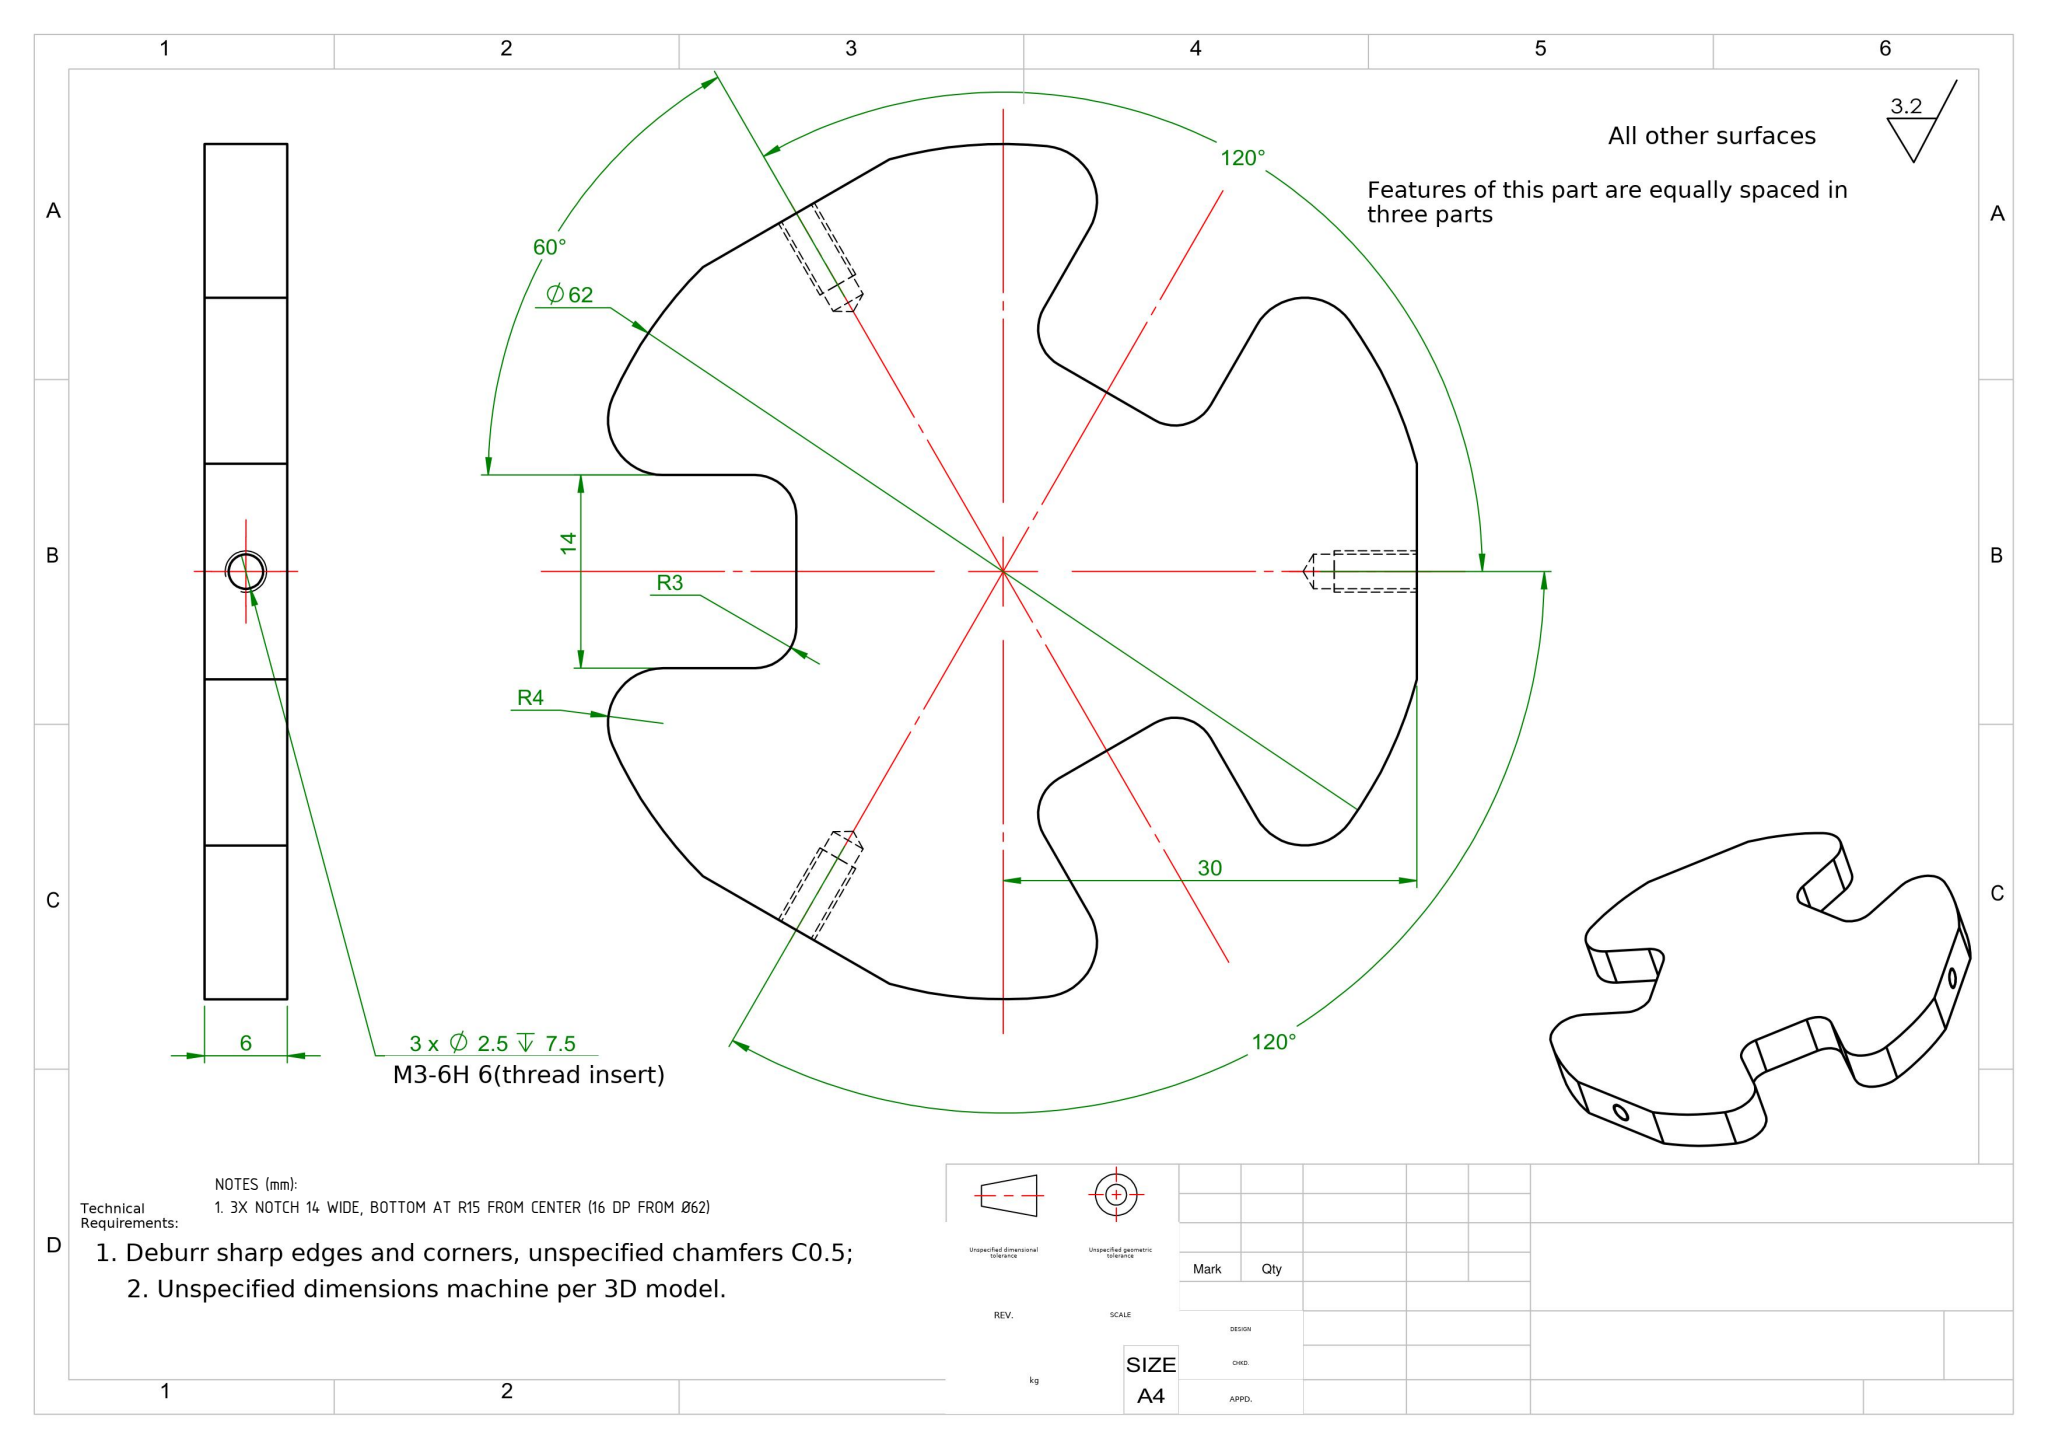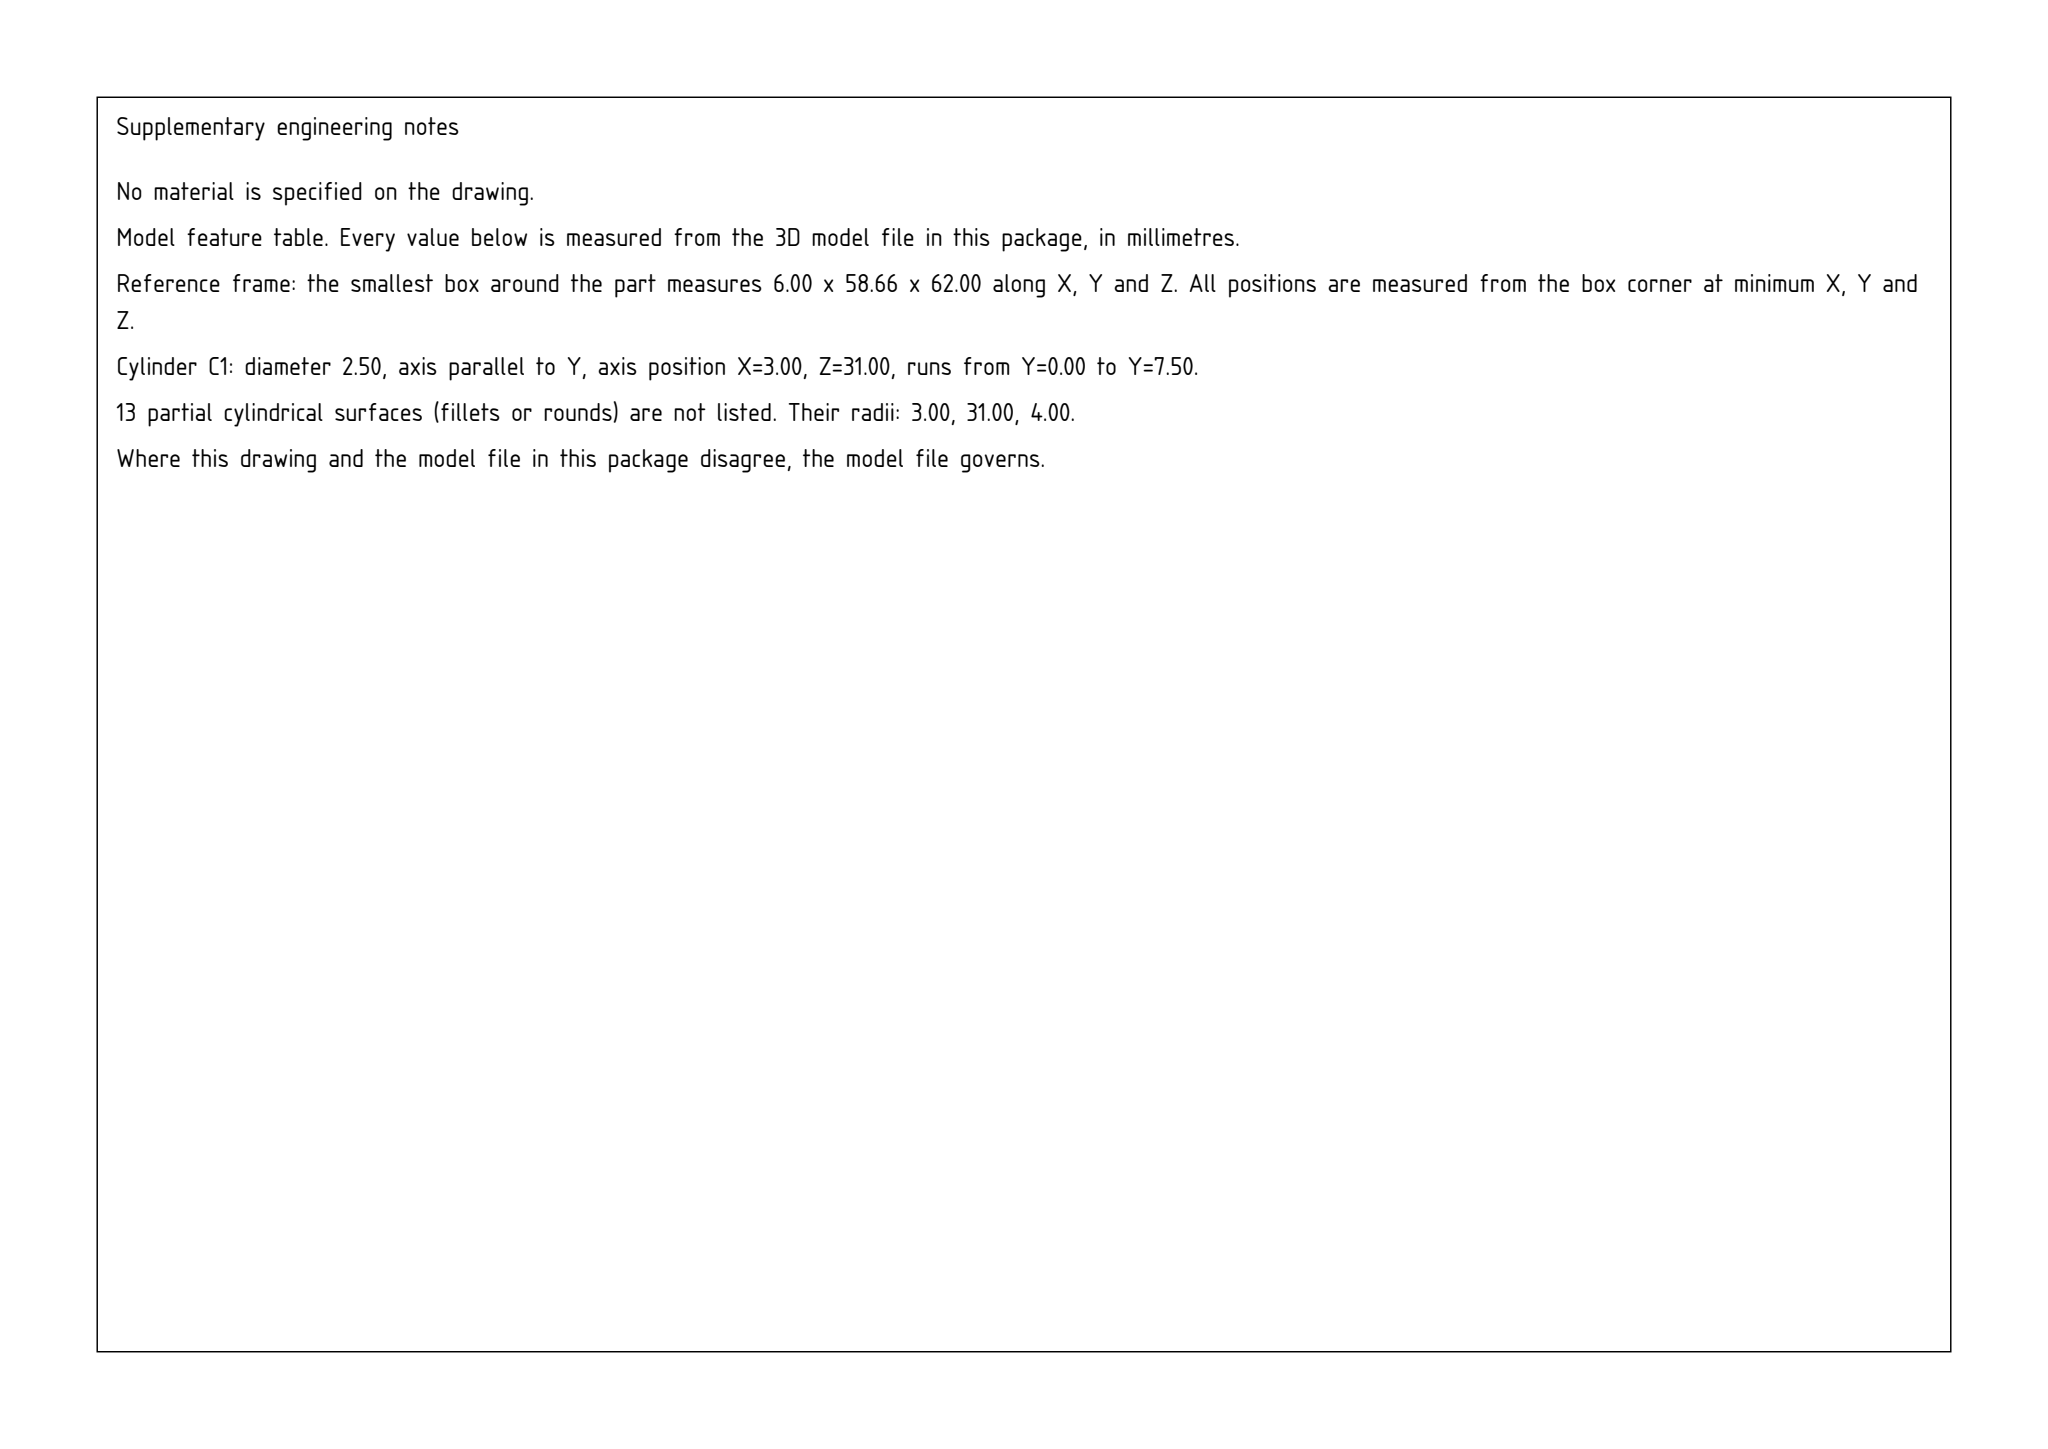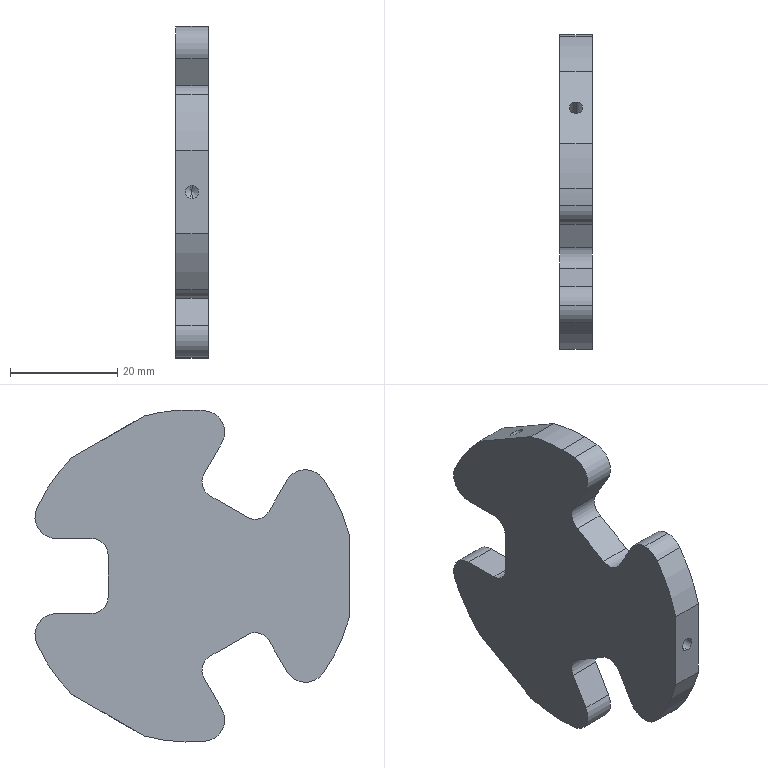Part | SolidWorks | mm | 1 solid | 47 faces | box 6 x 58.66 x 62 mm | volume 13645 mm3 | cylinder 27 | plane 14 | cone 6 | commonest cylinder face diameters 8 x7 6 x7 62 x7 2.5 x6
Drawing notes:
3X NOTCH 14 WIDE, BOTTOM AT R15 FROM CENTER (16 DP FROM Ø62) | from the solid: Planar face y=45 with Ø62 cyl axis at y=30, z=31: 45-30=R15; 31-15=16 deep